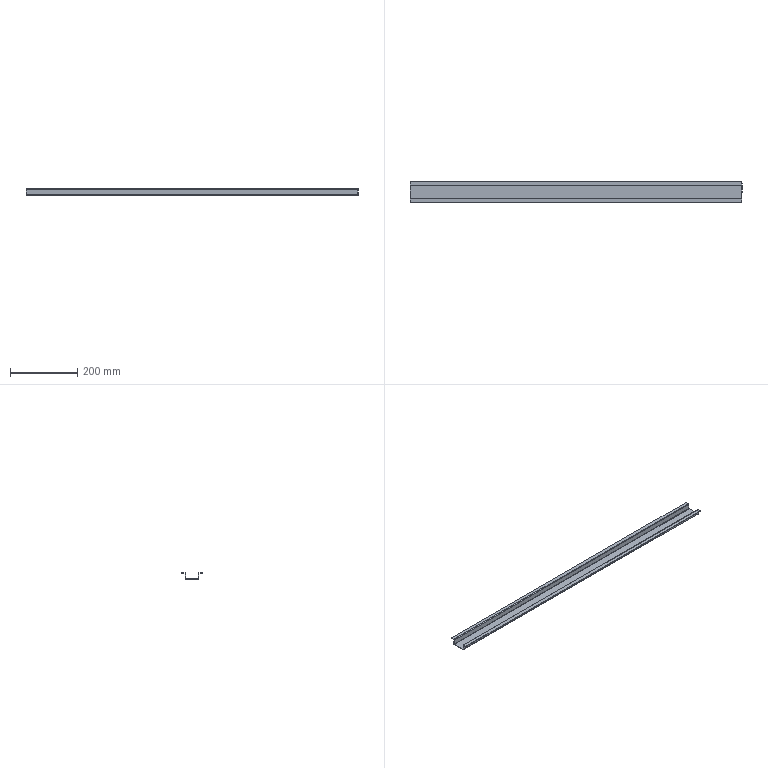Component | SolidWorks | AirFurnaceElectricalCabinet-DoorPanelAssembly-1_DoorPanelReinforcementPlate-L790-1 | 1 solid | 38 faces | box 990 x 61.6 x 18 mm | volume 110344 mm3 | plane 30 | cylinder 8 | commonest cylinder face diameters 3.9 x4 1.5 x4
STEP:
#1=CARTESIAN_POINT('',(-19.488,27.38,9.272));
#2=VERTEX_POINT('',#1);
#3=CARTESIAN_POINT('',(-19.488,28.801,9.272));
#4=VERTEX_POINT('',#3);
#5=CARTESIAN_POINT('',(-19.488,27.303,9.272));
#6=DIRECTION('',(0.,1.,0.));
#7=VECTOR('',#6,39.37);
#8=LINE('',#5,#7);
#9=EDGE_CURVE('',#2,#4,#8,.T.);
#10=ORIENTED_EDGE('',*,*,#9,.F.);
#11=CARTESIAN_POINT('',(-19.488,27.38,9.319));
#12=VERTEX_POINT('',#11);
#13=CARTESIAN_POINT('',(-19.488,27.38,9.272));
#14=DIRECTION('',(0.,-0.,1.));
#15=VECTOR('',#14,39.37);
#16=LINE('',#13,#15);
#17=EDGE_CURVE('',#2,#12,#16,.T.);
#18=ORIENTED_EDGE('',*,*,#17,.T.);
#19=CARTESIAN_POINT('',(-19.488,28.801,9.319));
#20=VERTEX_POINT('',#19);
#21=CARTESIAN_POINT('',(-19.488,27.303,9.319));
#22=DIRECTION('',(0.,1.,0.));
#23=VECTOR('',#22,39.37);
#24=LINE('',#21,#23);
#25=EDGE_CURVE('',#12,#20,#24,.T.);
#26=ORIENTED_EDGE('',*,*,#25,.T.);
#27=CARTESIAN_POINT('',(-19.488,28.801,9.319));
#28=DIRECTION('',(0.,0.,-1.));
#29=VECTOR('',#28,39.37);
#30=LINE('',#27,#29);
#31=EDGE_CURVE('',#20,#4,#30,.T.);
#32=ORIENTED_EDGE('',*,*,#31,.T.);
#33=EDGE_LOOP('',(#10,#18,#26,#32));
#34=FACE_OUTER_BOUND('',#33,.T.);
#35=CARTESIAN_POINT('',(-19.488,27.35,9.348));
#36=DIRECTION('',(-1.,0.,0.));
#37=DIRECTION('',(0.,1.,0.));
#38=AXIS2_PLACEMENT_3D('',#35,#36,#37);
#39=PLANE('',#38);
#40=ADVANCED_FACE('',(#34),#39,.T.);
#41=CARTESIAN_POINT('',(19.488,27.38,9.272));
#42=VERTEX_POINT('',#41);
#43=CARTESIAN_POINT('',(19.488,28.801,9.272));
#44=VERTEX_POINT('',#43);
#45=CARTESIAN_POINT('',(19.488,27.303,9.272));
#46=DIRECTION('',(0.,1.,0.));
#47=VECTOR('',#46,39.37);
#48=LINE('',#45,#47);
#49=EDGE_CURVE('',#42,#44,#48,.T.);
#50=ORIENTED_EDGE('',*,*,#49,.T.);
#51=CARTESIAN_POINT('',(19.488,28.801,9.319));
#52=VERTEX_POINT('',#51);
#53=CARTESIAN_POINT('',(19.488,28.801,9.272));
#54=DIRECTION('',(0.,-0.,1.));
#55=VECTOR('',#54,39.37);
#56=LINE('',#53,#55);
#57=EDGE_CURVE('',#44,#52,#56,.T.);
#58=ORIENTED_EDGE('',*,*,#57,.T.);
#59=CARTESIAN_POINT('',(19.488,27.38,9.319));
#60=VERTEX_POINT('',#59);
#61=CARTESIAN_POINT('',(19.488,27.303,9.319));
#62=DIRECTION('',(0.,1.,0.));
#63=VECTOR('',#62,39.37);
#64=LINE('',#61,#63);
#65=EDGE_CURVE('',#60,#52,#64,.T.);
#66=ORIENTED_EDGE('',*,*,#65,.F.);
#67=CARTESIAN_POINT('',(19.488,27.38,9.319));
#68=DIRECTION('',(0.,0.,-1.));
#69=VECTOR('',#68,39.37);
#70=LINE('',#67,#69);
#71=EDGE_CURVE('',#60,#42,#70,.T.);
#72=ORIENTED_EDGE('',*,*,#71,.T.);
#73=EDGE_LOOP('',(#50,#58,#66,#72));
#74=FACE_OUTER_BOUND('',#73,.T.);
#75=CARTESIAN_POINT('',(19.488,28.831,9.348));
#76=DIRECTION('',(1.,-0.,0.));
#77=DIRECTION('',(-0.,-1.,-0.));
#78=AXIS2_PLACEMENT_3D('',#75,#76,#77);
#79=PLANE('',#78);
#80=ADVANCED_FACE('',(#74),#79,.T.);
#81=ORIENTED_EDGE('',*,*,#49,.F.);
#82=CARTESIAN_POINT('',(-19.488,27.38,9.272));
#83=DIRECTION('',(1.,-0.,0.));
#84=VECTOR('',#83,39.37);
#85=LINE('',#82,#84);
#86=EDGE_CURVE('',#2,#42,#85,.T.);
#87=ORIENTED_EDGE('',*,*,#86,.F.);
#88=ORIENTED_EDGE('',*,*,#9,.T.);
#89=CARTESIAN_POINT('',(-19.488,28.801,9.272));
#90=DIRECTION('',(1.,-0.,0.));
#91=VECTOR('',#90,39.37);
#92=LINE('',#89,#91);
#93=EDGE_CURVE('',#4,#44,#92,.T.);
#94=ORIENTED_EDGE('',*,*,#93,.T.);
#95=EDGE_LOOP('',(#81,#87,#88,#94));
#96=FACE_OUTER_BOUND('',#95,.T.);
#97=CARTESIAN_POINT('',(-19.488,27.303,9.272));
#98=DIRECTION('',(0.,0.,-1.));
#99=DIRECTION('',(-0.,-1.,-0.));
#100=AXIS2_PLACEMENT_3D('',#97,#98,#99);
#101=PLANE('',#100);
#102=ADVANCED_FACE('',(#96),#101,.T.);
#103=ORIENTED_EDGE('',*,*,#65,.T.);
#104=CARTESIAN_POINT('',(-19.488,28.801,9.319));
#105=DIRECTION('',(1.,-0.,0.));
#106=VECTOR('',#105,39.37);
#107=LINE('',#104,#106);
#108=EDGE_CURVE('',#20,#52,#107,.T.);
#109=ORIENTED_EDGE('',*,*,#108,.F.);
#110=ORIENTED_EDGE('',*,*,#25,.F.);
#111=CARTESIAN_POINT('',(-19.488,27.38,9.319));
#112=DIRECTION('',(1.,-0.,0.));
#113=VECTOR('',#112,39.37);
#114=LINE('',#111,#113);
#115=EDGE_CURVE('',#12,#60,#114,.T.);
#116=ORIENTED_EDGE('',*,*,#115,.T.);
#117=EDGE_LOOP('',(#103,#109,#110,#116));
#118=FACE_OUTER_BOUND('',#117,.T.);
#119=CARTESIAN_POINT('',(-19.488,27.303,9.319));
#120=DIRECTION('',(0.,0.,-1.));
#121=DIRECTION('',(-0.,-1.,-0.));
#122=AXIS2_PLACEMENT_3D('',#119,#120,#121);
#123=PLANE('',#122);
#124=ADVANCED_FACE('',(#118),#123,.F.);
#125=ORIENTED_EDGE('',*,*,#31,.F.);
#126=CARTESIAN_POINT('',(-19.488,28.831,9.348));
#127=VERTEX_POINT('',#126);
#128=CARTESIAN_POINT('',(-19.488,28.801,9.348));
#129=DIRECTION('',(1.,-0.,0.));
#130=DIRECTION('',(0.,-1.,0.));
#131=AXIS2_PLACEMENT_3D('',#128,#129,#130);
#132=CIRCLE('',#131,0.02953);
#133=EDGE_CURVE('',#20,#127,#132,.T.);
#134=ORIENTED_EDGE('',*,*,#133,.T.);
#135=CARTESIAN_POINT('',(-19.488,28.878,9.348));
#136=VERTEX_POINT('',#135);
#137=CARTESIAN_POINT('',(-19.488,28.878,9.348));
#138=DIRECTION('',(-0.,-1.,-0.));
#139=VECTOR('',#138,39.37);
#140=LINE('',#137,#139);
#141=EDGE_CURVE('',#136,#127,#140,.T.);
#142=ORIENTED_EDGE('',*,*,#141,.F.);
#143=CARTESIAN_POINT('',(-19.488,28.801,9.348));
#144=DIRECTION('',(1.,-0.,0.));
#145=DIRECTION('',(0.,-1.,0.));
#146=AXIS2_PLACEMENT_3D('',#143,#144,#145);
#147=CIRCLE('',#146,0.07677);
#148=EDGE_CURVE('',#4,#136,#147,.T.);
#149=ORIENTED_EDGE('',*,*,#148,.F.);
#150=EDGE_LOOP('',(#125,#134,#142,#149));
#151=FACE_OUTER_BOUND('',#150,.T.);
#152=CARTESIAN_POINT('',(-19.488,28.801,9.348));
#153=DIRECTION('',(-1.,0.,0.));
#154=DIRECTION('',(0.,1.,0.));
#155=AXIS2_PLACEMENT_3D('',#152,#153,#154);
#156=PLANE('',#155);
#157=ADVANCED_FACE('',(#151),#156,.T.);
#158=CARTESIAN_POINT('',(19.488,28.831,9.348));
#159=VERTEX_POINT('',#158);
#160=CARTESIAN_POINT('',(19.488,28.878,9.348));
#161=VERTEX_POINT('',#160);
#162=CARTESIAN_POINT('',(19.488,28.831,9.348));
#163=DIRECTION('',(0.,1.,0.));
#164=VECTOR('',#163,39.37);
#165=LINE('',#162,#164);
#166=EDGE_CURVE('',#159,#161,#165,.T.);
#167=ORIENTED_EDGE('',*,*,#166,.F.);
#168=CARTESIAN_POINT('',(19.488,28.801,9.348));
#169=DIRECTION('',(-1.,0.,0.));
#170=DIRECTION('',(0.,-1.,0.));
#171=AXIS2_PLACEMENT_3D('',#168,#169,#170);
#172=CIRCLE('',#171,0.02953);
#173=EDGE_CURVE('',#159,#52,#172,.T.);
#174=ORIENTED_EDGE('',*,*,#173,.T.);
#175=ORIENTED_EDGE('',*,*,#57,.F.);
#176=CARTESIAN_POINT('',(19.488,28.801,9.348));
#177=DIRECTION('',(-1.,0.,0.));
#178=DIRECTION('',(0.,1.,0.));
#179=AXIS2_PLACEMENT_3D('',#176,#177,#178);
#180=CIRCLE('',#179,0.07677);
#181=EDGE_CURVE('',#161,#44,#180,.T.);
#182=ORIENTED_EDGE('',*,*,#181,.F.);
#183=EDGE_LOOP('',(#167,#174,#175,#182));
#184=FACE_OUTER_BOUND('',#183,.T.);
#185=CARTESIAN_POINT('',(19.488,28.801,9.348));
#186=DIRECTION('',(1.,-0.,0.));
#187=DIRECTION('',(-0.,-1.,-0.));
#188=AXIS2_PLACEMENT_3D('',#185,#186,#187);
#189=PLANE('',#188);
#190=ADVANCED_FACE('',(#184),#189,.T.);
#191=ORIENTED_EDGE('',*,*,#181,.T.);
#192=ORIENTED_EDGE('',*,*,#93,.F.);
#193=ORIENTED_EDGE('',*,*,#148,.T.);
#194=CARTESIAN_POINT('',(-19.488,28.878,9.348));
#195=DIRECTION('',(1.,-0.,0.));
#196=VECTOR('',#195,39.37);
#197=LINE('',#194,#196);
#198=EDGE_CURVE('',#136,#161,#197,.T.);
#199=ORIENTED_EDGE('',*,*,#198,.T.);
#200=EDGE_LOOP('',(#191,#192,#193,#199));
#201=FACE_OUTER_BOUND('',#200,.T.);
#202=CARTESIAN_POINT('',(-38.976,28.801,9.348));
#203=DIRECTION('',(1.,-0.,0.));
#204=DIRECTION('',(0.,-1.,0.));
#205=AXIS2_PLACEMENT_3D('',#202,#203,#204);
#206=CYLINDRICAL_SURFACE('',#205,0.07677);
#207=ADVANCED_FACE('',(#201),#206,.T.);
#208=ORIENTED_EDGE('',*,*,#173,.F.);
#209=CARTESIAN_POINT('',(-19.488,28.831,9.348));
#210=DIRECTION('',(1.,-0.,0.));
#211=VECTOR('',#210,39.37);
#212=LINE('',#209,#211);
#213=EDGE_CURVE('',#127,#159,#212,.T.);
#214=ORIENTED_EDGE('',*,*,#213,.F.);
#215=ORIENTED_EDGE('',*,*,#133,.F.);
#216=ORIENTED_EDGE('',*,*,#108,.T.);
#217=EDGE_LOOP('',(#208,#214,#215,#216));
#218=FACE_OUTER_BOUND('',#217,.T.);
#219=CARTESIAN_POINT('',(-38.976,28.801,9.348));
#220=DIRECTION('',(1.,-0.,0.));
#221=DIRECTION('',(0.,-1.,0.));
#222=AXIS2_PLACEMENT_3D('',#219,#220,#221);
#223=CYLINDRICAL_SURFACE('',#222,0.02953);
#224=ADVANCED_FACE('',(#218),#223,.F.);
#225=CARTESIAN_POINT('',(19.488,29.303,9.933));
#226=VERTEX_POINT('',#225);
#227=CARTESIAN_POINT('',(19.488,29.303,9.98));
#228=VERTEX_POINT('',#227);
#229=CARTESIAN_POINT('',(19.488,29.303,9.933));
#230=DIRECTION('',(0.,-0.,1.));
#231=VECTOR('',#230,39.37);
#232=LINE('',#229,#231);
#233=EDGE_CURVE('',#226,#228,#232,.T.);
#234=ORIENTED_EDGE('',*,*,#233,.F.);
#235=CARTESIAN_POINT('',(-19.488,29.303,9.933));
#236=VERTEX_POINT('',#235);
#237=CARTESIAN_POINT('',(-19.488,29.303,9.933));
#238=DIRECTION('',(1.,-0.,0.));
#239=VECTOR('',#238,39.37);
#240=LINE('',#237,#239);
#241=EDGE_CURVE('',#236,#226,#240,.T.);
#242=ORIENTED_EDGE('',*,*,#241,.F.);
#243=CARTESIAN_POINT('',(-19.488,29.303,9.98));
#244=VERTEX_POINT('',#243);
#245=CARTESIAN_POINT('',(-19.488,29.303,9.933));
#246=DIRECTION('',(0.,-0.,1.));
#247=VECTOR('',#246,39.37);
#248=LINE('',#245,#247);
#249=EDGE_CURVE('',#236,#244,#248,.T.);
#250=ORIENTED_EDGE('',*,*,#249,.T.);
#251=CARTESIAN_POINT('',(-19.488,29.303,9.98));
#252=DIRECTION('',(1.,-0.,0.));
#253=VECTOR('',#252,39.37);
#254=LINE('',#251,#253);
#255=EDGE_CURVE('',#244,#228,#254,.T.);
#256=ORIENTED_EDGE('',*,*,#255,.T.);
#257=EDGE_LOOP('',(#234,#242,#250,#256));
#258=FACE_OUTER_BOUND('',#257,.T.);
#259=CARTESIAN_POINT('',(-19.488,29.303,9.933));
#260=DIRECTION('',(0.,1.,0.));
#261=DIRECTION('',(1.,-0.,0.));
#262=AXIS2_PLACEMENT_3D('',#259,#260,#261);
#263=PLANE('',#262);
#264=ADVANCED_FACE('',(#258),#263,.T.);
#265=CARTESIAN_POINT('',(19.488,28.907,9.98));
#266=VERTEX_POINT('',#265);
#267=CARTESIAN_POINT('',(19.488,28.878,9.98));
#268=DIRECTION('',(0.,1.,0.));
#269=VECTOR('',#268,39.37);
#270=LINE('',#267,#269);
#271=EDGE_CURVE('',#266,#228,#270,.T.);
#272=ORIENTED_EDGE('',*,*,#271,.F.);
#273=CARTESIAN_POINT('',(19.488,28.907,9.933));
#274=VERTEX_POINT('',#273);
#275=CARTESIAN_POINT('',(19.488,28.907,9.98));
#276=DIRECTION('',(0.,0.,-1.));
#277=VECTOR('',#276,39.37);
#278=LINE('',#275,#277);
#279=EDGE_CURVE('',#266,#274,#278,.T.);
#280=ORIENTED_EDGE('',*,*,#279,.T.);
#281=CARTESIAN_POINT('',(19.488,28.878,9.933));
#282=DIRECTION('',(0.,1.,0.));
#283=VECTOR('',#282,39.37);
#284=LINE('',#281,#283);
#285=EDGE_CURVE('',#274,#226,#284,.T.);
#286=ORIENTED_EDGE('',*,*,#285,.T.);
#287=ORIENTED_EDGE('',*,*,#233,.T.);
#288=EDGE_LOOP('',(#272,#280,#286,#287));
#289=FACE_OUTER_BOUND('',#288,.T.);
#290=CARTESIAN_POINT('',(19.488,28.907,9.904));
#291=DIRECTION('',(1.,-0.,0.));
#292=DIRECTION('',(-0.,-1.,-0.));
#293=AXIS2_PLACEMENT_3D('',#290,#291,#292);
#294=PLANE('',#293);
#295=ADVANCED_FACE('',(#289),#294,.T.);
#296=ORIENTED_EDGE('',*,*,#271,.T.);
#297=ORIENTED_EDGE('',*,*,#255,.F.);
#298=CARTESIAN_POINT('',(-19.488,28.907,9.98));
#299=VERTEX_POINT('',#298);
#300=CARTESIAN_POINT('',(-19.488,28.878,9.98));
#301=DIRECTION('',(0.,1.,0.));
#302=VECTOR('',#301,39.37);
#303=LINE('',#300,#302);
#304=EDGE_CURVE('',#299,#244,#303,.T.);
#305=ORIENTED_EDGE('',*,*,#304,.F.);
#306=CARTESIAN_POINT('',(-19.488,28.907,9.98));
#307=DIRECTION('',(1.,-0.,0.));
#308=VECTOR('',#307,39.37);
#309=LINE('',#306,#308);
#310=EDGE_CURVE('',#299,#266,#309,.T.);
#311=ORIENTED_EDGE('',*,*,#310,.T.);
#312=EDGE_LOOP('',(#296,#297,#305,#311));
#313=FACE_OUTER_BOUND('',#312,.T.);
#314=CARTESIAN_POINT('',(-19.488,28.878,9.98));
#315=DIRECTION('',(0.,0.,-1.));
#316=DIRECTION('',(-0.,-1.,-0.));
#317=AXIS2_PLACEMENT_3D('',#314,#315,#316);
#318=PLANE('',#317);
#319=ADVANCED_FACE('',(#313),#318,.F.);
#320=CARTESIAN_POINT('',(-19.488,28.907,9.933));
#321=VERTEX_POINT('',#320);
#322=CARTESIAN_POINT('',(-19.488,28.878,9.933));
#323=DIRECTION('',(0.,1.,0.));
#324=VECTOR('',#323,39.37);
#325=LINE('',#322,#324);
#326=EDGE_CURVE('',#321,#236,#325,.T.);
#327=ORIENTED_EDGE('',*,*,#326,.F.);
#328=CARTESIAN_POINT('',(-19.488,28.907,9.933));
#329=DIRECTION('',(0.,-0.,1.));
#330=VECTOR('',#329,39.37);
#331=LINE('',#328,#330);
#332=EDGE_CURVE('',#321,#299,#331,.T.);
#333=ORIENTED_EDGE('',*,*,#332,.T.);
#334=ORIENTED_EDGE('',*,*,#304,.T.);
#335=ORIENTED_EDGE('',*,*,#249,.F.);
#336=EDGE_LOOP('',(#327,#333,#334,#335));
#337=FACE_OUTER_BOUND('',#336,.T.);
#338=CARTESIAN_POINT('',(-19.488,28.831,9.904));
#339=DIRECTION('',(-1.,0.,0.));
#340=DIRECTION('',(0.,1.,0.));
#341=AXIS2_PLACEMENT_3D('',#338,#339,#340);
#342=PLANE('',#341);
#343=ADVANCED_FACE('',(#337),#342,.T.);
#344=ORIENTED_EDGE('',*,*,#285,.F.);
#345=CARTESIAN_POINT('',(-19.488,28.907,9.933));
#346=DIRECTION('',(1.,-0.,0.));
#347=VECTOR('',#346,39.37);
#348=LINE('',#345,#347);
#349=EDGE_CURVE('',#321,#274,#348,.T.);
#350=ORIENTED_EDGE('',*,*,#349,.F.);
#351=ORIENTED_EDGE('',*,*,#326,.T.);
#352=ORIENTED_EDGE('',*,*,#241,.T.);
#353=EDGE_LOOP('',(#344,#350,#351,#352));
#354=FACE_OUTER_BOUND('',#353,.T.);
#355=CARTESIAN_POINT('',(-19.488,28.878,9.933));
#356=DIRECTION('',(0.,0.,-1.));
#357=DIRECTION('',(-0.,-1.,-0.));
#358=AXIS2_PLACEMENT_3D('',#355,#356,#357);
#359=PLANE('',#358);
#360=ADVANCED_FACE('',(#354),#359,.T.);
#361=ORIENTED_EDGE('',*,*,#279,.F.);
#362=CARTESIAN_POINT('',(19.488,28.831,9.904));
#363=VERTEX_POINT('',#362);
#364=CARTESIAN_POINT('',(19.488,28.907,9.904));
#365=DIRECTION('',(1.,-0.,0.));
#366=DIRECTION('',(0.,0.,-1.));
#367=AXIS2_PLACEMENT_3D('',#364,#365,#366);
#368=CIRCLE('',#367,0.07677);
#369=EDGE_CURVE('',#266,#363,#368,.T.);
#370=ORIENTED_EDGE('',*,*,#369,.T.);
#371=CARTESIAN_POINT('',(19.488,28.878,9.904));
#372=VERTEX_POINT('',#371);
#373=CARTESIAN_POINT('',(19.488,28.878,9.904));
#374=DIRECTION('',(-0.,-1.,-0.));
#375=VECTOR('',#374,39.37);
#376=LINE('',#373,#375);
#377=EDGE_CURVE('',#372,#363,#376,.T.);
#378=ORIENTED_EDGE('',*,*,#377,.F.);
#379=CARTESIAN_POINT('',(19.488,28.907,9.904));
#380=DIRECTION('',(1.,-0.,0.));
#381=DIRECTION('',(0.,0.,-1.));
#382=AXIS2_PLACEMENT_3D('',#379,#380,#381);
#383=CIRCLE('',#382,0.02953);
#384=EDGE_CURVE('',#274,#372,#383,.T.);
#385=ORIENTED_EDGE('',*,*,#384,.F.);
#386=EDGE_LOOP('',(#361,#370,#378,#385));
#387=FACE_OUTER_BOUND('',#386,.T.);
#388=CARTESIAN_POINT('',(19.488,28.907,9.904));
#389=DIRECTION('',(-1.,0.,0.));
#390=DIRECTION('',(0.,0.,1.));
#391=AXIS2_PLACEMENT_3D('',#388,#389,#390);
#392=PLANE('',#391);
#393=ADVANCED_FACE('',(#387),#392,.F.);
#394=ORIENTED_EDGE('',*,*,#369,.F.);
#395=ORIENTED_EDGE('',*,*,#310,.F.);
#396=CARTESIAN_POINT('',(-19.488,28.831,9.904));
#397=VERTEX_POINT('',#396);
#398=CARTESIAN_POINT('',(-19.488,28.907,9.904));
#399=DIRECTION('',(-1.,0.,0.));
#400=DIRECTION('',(0.,0.,-1.));
#401=AXIS2_PLACEMENT_3D('',#398,#399,#400);
#402=CIRCLE('',#401,0.07677);
#403=EDGE_CURVE('',#397,#299,#402,.T.);
#404=ORIENTED_EDGE('',*,*,#403,.F.);
#405=CARTESIAN_POINT('',(-19.488,28.831,9.904));
#406=DIRECTION('',(1.,-0.,0.));
#407=VECTOR('',#406,39.37);
#408=LINE('',#405,#407);
#409=EDGE_CURVE('',#397,#363,#408,.T.);
#410=ORIENTED_EDGE('',*,*,#409,.T.);
#411=EDGE_LOOP('',(#394,#395,#404,#410));
#412=FACE_OUTER_BOUND('',#411,.T.);
#413=CARTESIAN_POINT('',(-38.976,28.907,9.904));
#414=DIRECTION('',(1.,-0.,0.));
#415=DIRECTION('',(0.,0.,-1.));
#416=AXIS2_PLACEMENT_3D('',#413,#414,#415);
#417=CYLINDRICAL_SURFACE('',#416,0.07677);
#418=ADVANCED_FACE('',(#412),#417,.T.);
#419=CARTESIAN_POINT('',(-19.488,28.878,9.904));
#420=VERTEX_POINT('',#419);
#421=CARTESIAN_POINT('',(-19.488,28.831,9.904));
#422=DIRECTION('',(0.,1.,0.));
#423=VECTOR('',#422,39.37);
#424=LINE('',#421,#423);
#425=EDGE_CURVE('',#397,#420,#424,.T.);
#426=ORIENTED_EDGE('',*,*,#425,.F.);
#427=ORIENTED_EDGE('',*,*,#403,.T.);
#428=ORIENTED_EDGE('',*,*,#332,.F.);
#429=CARTESIAN_POINT('',(-19.488,28.907,9.904));
#430=DIRECTION('',(-1.,0.,0.));
#431=DIRECTION('',(0.,0.,1.));
#432=AXIS2_PLACEMENT_3D('',#429,#430,#431);
#433=CIRCLE('',#432,0.02953);
#434=EDGE_CURVE('',#420,#321,#433,.T.);
#435=ORIENTED_EDGE('',*,*,#434,.F.);
#436=EDGE_LOOP('',(#426,#427,#428,#435));
#437=FACE_OUTER_BOUND('',#436,.T.);
#438=CARTESIAN_POINT('',(-19.488,28.907,9.904));
#439=DIRECTION('',(1.,-0.,-0.));
#440=DIRECTION('',(-0.,-0.,-1.));
#441=AXIS2_PLACEMENT_3D('',#438,#439,#440);
#442=PLANE('',#441);
#443=ADVANCED_FACE('',(#437),#442,.F.);
#444=ORIENTED_EDGE('',*,*,#384,.T.);
#445=CARTESIAN_POINT('',(-19.488,28.878,9.904));
#446=DIRECTION('',(1.,-0.,0.));
#447=VECTOR('',#446,39.37);
#448=LINE('',#445,#447);
#449=EDGE_CURVE('',#420,#372,#448,.T.);
#450=ORIENTED_EDGE('',*,*,#449,.F.);
#451=ORIENTED_EDGE('',*,*,#434,.T.);
#452=ORIENTED_EDGE('',*,*,#349,.T.);
#453=EDGE_LOOP('',(#444,#450,#451,#452));
#454=FACE_OUTER_BOUND('',#453,.T.);
#455=CARTESIAN_POINT('',(-38.976,28.907,9.904));
#456=DIRECTION('',(1.,-0.,0.));
#457=DIRECTION('',(0.,0.,-1.));
#458=AXIS2_PLACEMENT_3D('',#455,#456,#457);
#459=CYLINDRICAL_SURFACE('',#458,0.02953);
#460=ADVANCED_FACE('',(#454),#459,.F.);
#461=CARTESIAN_POINT('',(19.488,28.878,9.272));
#462=DIRECTION('',(0.,-0.,1.));
#463=VECTOR('',#462,39.37);
#464=LINE('',#461,#463);
#465=EDGE_CURVE('',#161,#372,#464,.T.);
#466=ORIENTED_EDGE('',*,*,#465,.F.);
#467=ORIENTED_EDGE('',*,*,#198,.F.);
#468=CARTESIAN_POINT('',(-19.488,28.878,9.272));
#469=DIRECTION('',(0.,-0.,1.));
#470=VECTOR('',#469,39.37);
#471=LINE('',#468,#470);
#472=EDGE_CURVE('',#136,#420,#471,.T.);
#473=ORIENTED_EDGE('',*,*,#472,.T.);
#474=ORIENTED_EDGE('',*,*,#449,.T.);
#475=EDGE_LOOP('',(#466,#467,#473,#474));
#476=FACE_OUTER_BOUND('',#475,.T.);
#477=CARTESIAN_POINT('',(-19.488,28.878,9.272));
#478=DIRECTION('',(0.,1.,0.));
#479=DIRECTION('',(1.,-0.,0.));
#480=AXIS2_PLACEMENT_3D('',#477,#478,#479);
#481=PLANE('',#480);
#482=ADVANCED_FACE('',(#476),#481,.T.);
#483=ORIENTED_EDGE('',*,*,#472,.F.);
#484=ORIENTED_EDGE('',*,*,#141,.T.);
#485=CARTESIAN_POINT('',(-19.488,28.831,9.272));
#486=DIRECTION('',(0.,-0.,1.));
#487=VECTOR('',#486,39.37);
#488=LINE('',#485,#487);
#489=EDGE_CURVE('',#127,#397,#488,.T.);
#490=ORIENTED_EDGE('',*,*,#489,.T.);
#491=ORIENTED_EDGE('',*,*,#425,.T.);
#492=EDGE_LOOP('',(#483,#484,#490,#491));
#493=FACE_OUTER_BOUND('',#492,.T.);
#494=CARTESIAN_POINT('',(-19.488,28.801,9.319));
#495=DIRECTION('',(-1.,0.,0.));
#496=DIRECTION('',(0.,1.,0.));
#497=AXIS2_PLACEMENT_3D('',#494,#495,#496);
#498=PLANE('',#497);
#499=ADVANCED_FACE('',(#493),#498,.T.);
#500=CARTESIAN_POINT('',(19.488,28.831,9.272));
#501=DIRECTION('',(0.,-0.,1.));
#502=VECTOR('',#501,39.37);
#503=LINE('',#500,#502);
#504=EDGE_CURVE('',#159,#363,#503,.T.);
#505=ORIENTED_EDGE('',*,*,#504,.T.);
#506=ORIENTED_EDGE('',*,*,#409,.F.);
#507=ORIENTED_EDGE('',*,*,#489,.F.);
#508=ORIENTED_EDGE('',*,*,#213,.T.);
#509=EDGE_LOOP('',(#505,#506,#507,#508));
#510=FACE_OUTER_BOUND('',#509,.T.);
#511=CARTESIAN_POINT('',(-19.488,28.831,9.272));
#512=DIRECTION('',(0.,1.,0.));
#513=DIRECTION('',(1.,-0.,0.));
#514=AXIS2_PLACEMENT_3D('',#511,#512,#513);
#515=PLANE('',#514);
#516=ADVANCED_FACE('',(#510),#515,.F.);
#517=ORIENTED_EDGE('',*,*,#465,.T.);
#518=ORIENTED_EDGE('',*,*,#377,.T.);
#519=ORIENTED_EDGE('',*,*,#504,.F.);
#520=ORIENTED_EDGE('',*,*,#166,.T.);
#521=EDGE_LOOP('',(#517,#518,#519,#520));
#522=FACE_OUTER_BOUND('',#521,.T.);
#523=CARTESIAN_POINT('',(19.488,28.907,9.98));
#524=DIRECTION('',(1.,-0.,0.));
#525=DIRECTION('',(-0.,-1.,-0.));
#526=AXIS2_PLACEMENT_3D('',#523,#524,#525);
#527=PLANE('',#526);
#528=ADVANCED_FACE('',(#522),#527,.T.);
#529=CARTESIAN_POINT('',(-19.488,27.35,9.348));
#530=VERTEX_POINT('',#529);
#531=CARTESIAN_POINT('',(-19.488,27.303,9.348));
#532=VERTEX_POINT('',#531);
#533=CARTESIAN_POINT('',(-19.488,27.35,9.348));
#534=DIRECTION('',(-0.,-1.,-0.));
#535=VECTOR('',#534,39.37);
#536=LINE('',#533,#535);
#537=EDGE_CURVE('',#530,#532,#536,.T.);
#538=ORIENTED_EDGE('',*,*,#537,.F.);
#539=CARTESIAN_POINT('',(-19.488,27.38,9.348));
#540=DIRECTION('',(1.,-0.,0.));
#541=DIRECTION('',(0.,1.,0.));
#542=AXIS2_PLACEMENT_3D('',#539,#540,#541);
#543=CIRCLE('',#542,0.02953);
#544=EDGE_CURVE('',#530,#12,#543,.T.);
#545=ORIENTED_EDGE('',*,*,#544,.T.);
#546=ORIENTED_EDGE('',*,*,#17,.F.);
#547=CARTESIAN_POINT('',(-19.488,27.38,9.348));
#548=DIRECTION('',(1.,-0.,0.));
#549=DIRECTION('',(0.,-1.,0.));
#550=AXIS2_PLACEMENT_3D('',#547,#548,#549);
#551=CIRCLE('',#550,0.07677);
#552=EDGE_CURVE('',#532,#2,#551,.T.);
#553=ORIENTED_EDGE('',*,*,#552,.F.);
#554=EDGE_LOOP('',(#538,#545,#546,#553));
#555=FACE_OUTER_BOUND('',#554,.T.);
#556=CARTESIAN_POINT('',(-19.488,27.38,9.348));
#557=DIRECTION('',(-1.,0.,0.));
#558=DIRECTION('',(0.,1.,0.));
#559=AXIS2_PLACEMENT_3D('',#556,#557,#558);
#560=PLANE('',#559);
#561=ADVANCED_FACE('',(#555),#560,.T.);
#562=ORIENTED_EDGE('',*,*,#71,.F.);
#563=CARTESIAN_POINT('',(19.488,27.35,9.348));
#564=VERTEX_POINT('',#563);
#565=CARTESIAN_POINT('',(19.488,27.38,9.348));
#566=DIRECTION('',(-1.,0.,0.));
#567=DIRECTION('',(0.,1.,0.));
#568=AXIS2_PLACEMENT_3D('',#565,#566,#567);
#569=CIRCLE('',#568,0.02953);
#570=EDGE_CURVE('',#60,#564,#569,.T.);
#571=ORIENTED_EDGE('',*,*,#570,.T.);
#572=CARTESIAN_POINT('',(19.488,27.303,9.348));
#573=VERTEX_POINT('',#572);
#574=CARTESIAN_POINT('',(19.488,27.303,9.348));
#575=DIRECTION('',(0.,1.,0.));
#576=VECTOR('',#575,39.37);
#577=LINE('',#574,#576);
#578=EDGE_CURVE('',#573,#564,#577,.T.);
#579=ORIENTED_EDGE('',*,*,#578,.F.);
#580=CARTESIAN_POINT('',(19.488,27.38,9.348));
#581=DIRECTION('',(-1.,0.,0.));
#582=DIRECTION('',(0.,1.,0.));
#583=AXIS2_PLACEMENT_3D('',#580,#581,#582);
#584=CIRCLE('',#583,0.07677);
#585=EDGE_CURVE('',#42,#573,#584,.T.);
#586=ORIENTED_EDGE('',*,*,#585,.F.);
#587=EDGE_LOOP('',(#562,#571,#579,#586));
#588=FACE_OUTER_BOUND('',#587,.T.);
#589=CARTESIAN_POINT('',(19.488,27.38,9.348));
#590=DIRECTION('',(1.,-0.,0.));
#591=DIRECTION('',(-0.,-1.,-0.));
#592=AXIS2_PLACEMENT_3D('',#589,#590,#591);
#593=PLANE('',#592);
#594=ADVANCED_FACE('',(#588),#593,.T.);
#595=ORIENTED_EDGE('',*,*,#585,.T.);
#596=CARTESIAN_POINT('',(-19.488,27.303,9.348));
#597=DIRECTION('',(1.,-0.,0.));
#598=VECTOR('',#597,39.37);
#599=LINE('',#596,#598);
#600=EDGE_CURVE('',#532,#573,#599,.T.);
#601=ORIENTED_EDGE('',*,*,#600,.F.);
#602=ORIENTED_EDGE('',*,*,#552,.T.);
#603=ORIENTED_EDGE('',*,*,#86,.T.);
#604=EDGE_LOOP('',(#595,#601,#602,#603));
#605=FACE_OUTER_BOUND('',#604,.T.);
#606=CARTESIAN_POINT('',(38.976,27.38,9.348));
#607=DIRECTION('',(-1.,0.,0.));
#608=DIRECTION('',(0.,1.,0.));
#609=AXIS2_PLACEMENT_3D('',#606,#607,#608);
#610=CYLINDRICAL_SURFACE('',#609,0.07677);
#611=ADVANCED_FACE('',(#605),#610,.T.);
#612=ORIENTED_EDGE('',*,*,#570,.F.);
#613=ORIENTED_EDGE('',*,*,#115,.F.);
#614=ORIENTED_EDGE('',*,*,#544,.F.);
#615=CARTESIAN_POINT('',(-19.488,27.35,9.348));
#616=DIRECTION('',(1.,-0.,0.));
#617=VECTOR('',#616,39.37);
#618=LINE('',#615,#617);
#619=EDGE_CURVE('',#530,#564,#618,.T.);
#620=ORIENTED_EDGE('',*,*,#619,.T.);
#621=EDGE_LOOP('',(#612,#613,#614,#620));
#622=FACE_OUTER_BOUND('',#621,.T.);
#623=CARTESIAN_POINT('',(38.976,27.38,9.348));
#624=DIRECTION('',(-1.,0.,0.));
#625=DIRECTION('',(0.,1.,0.));
#626=AXIS2_PLACEMENT_3D('',#623,#624,#625);
#627=CYLINDRICAL_SURFACE('',#626,0.02953);
#628=ADVANCED_FACE('',(#622),#627,.F.);
#629=CARTESIAN_POINT('',(19.488,27.303,9.904));
#630=VERTEX_POINT('',#629);
#631=CARTESIAN_POINT('',(19.488,27.303,9.933));
#632=DIRECTION('',(0.,0.,-1.));
#633=VECTOR('',#632,39.37);
#634=LINE('',#631,#633);
#635=EDGE_CURVE('',#630,#573,#634,.T.);
#636=ORIENTED_EDGE('',*,*,#635,.F.);
#637=CARTESIAN_POINT('',(-19.488,27.303,9.904));
#638=VERTEX_POINT('',#637);
#639=CARTESIAN_POINT('',(-19.488,27.303,9.904));
#640=DIRECTION('',(1.,-0.,0.));
#641=VECTOR('',#640,39.37);
#642=LINE('',#639,#641);
#643=EDGE_CURVE('',#638,#630,#642,.T.);
#644=ORIENTED_EDGE('',*,*,#643,.F.);
#645=CARTESIAN_POINT('',(-19.488,27.303,9.933));
#646=DIRECTION('',(0.,0.,-1.));
#647=VECTOR('',#646,39.37);
#648=LINE('',#645,#647);
#649=EDGE_CURVE('',#638,#532,#648,.T.);
#650=ORIENTED_EDGE('',*,*,#649,.T.);
#651=ORIENTED_EDGE('',*,*,#600,.T.);
#652=EDGE_LOOP('',(#636,#644,#650,#651));
#653=FACE_OUTER_BOUND('',#652,.T.);
#654=CARTESIAN_POINT('',(-19.488,27.303,9.933));
#655=DIRECTION('',(-0.,-1.,-0.));
#656=DIRECTION('',(-1.,0.,0.));
#657=AXIS2_PLACEMENT_3D('',#654,#655,#656);
#658=PLANE('',#657);
#659=ADVANCED_FACE('',(#653),#658,.T.);
#660=ORIENTED_EDGE('',*,*,#635,.T.);
#661=ORIENTED_EDGE('',*,*,#578,.T.);
#662=CARTESIAN_POINT('',(19.488,27.35,9.904));
#663=VERTEX_POINT('',#662);
#664=CARTESIAN_POINT('',(19.488,27.35,9.933));
#665=DIRECTION('',(0.,0.,-1.));
#666=VECTOR('',#665,39.37);
#667=LINE('',#664,#666);
#668=EDGE_CURVE('',#663,#564,#667,.T.);
#669=ORIENTED_EDGE('',*,*,#668,.F.);
#670=CARTESIAN_POINT('',(19.488,27.35,9.904));
#671=DIRECTION('',(-0.,-1.,-0.));
#672=VECTOR('',#671,39.37);
#673=LINE('',#670,#672);
#674=EDGE_CURVE('',#663,#630,#673,.T.);
#675=ORIENTED_EDGE('',*,*,#674,.T.);
#676=EDGE_LOOP('',(#660,#661,#669,#675));
#677=FACE_OUTER_BOUND('',#676,.T.);
#678=CARTESIAN_POINT('',(19.488,27.38,9.319));
#679=DIRECTION('',(1.,-0.,0.));
#680=DIRECTION('',(-0.,-1.,-0.));
#681=AXIS2_PLACEMENT_3D('',#678,#679,#680);
#682=PLANE('',#681);
#683=ADVANCED_FACE('',(#677),#682,.T.);
#684=ORIENTED_EDGE('',*,*,#668,.T.);
#685=ORIENTED_EDGE('',*,*,#619,.F.);
#686=CARTESIAN_POINT('',(-19.488,27.35,9.904));
#687=VERTEX_POINT('',#686);
#688=CARTESIAN_POINT('',(-19.488,27.35,9.933));
#689=DIRECTION('',(0.,0.,-1.));
#690=VECTOR('',#689,39.37);
#691=LINE('',#688,#690);
#692=EDGE_CURVE('',#687,#530,#691,.T.);
#693=ORIENTED_EDGE('',*,*,#692,.F.);
#694=CARTESIAN_POINT('',(-19.488,27.35,9.904));
#695=DIRECTION('',(1.,-0.,0.));
#696=VECTOR('',#695,39.37);
#697=LINE('',#694,#696);
#698=EDGE_CURVE('',#687,#663,#697,.T.);
#699=ORIENTED_EDGE('',*,*,#698,.T.);
#700=EDGE_LOOP('',(#684,#685,#693,#699));
#701=FACE_OUTER_BOUND('',#700,.T.);
#702=CARTESIAN_POINT('',(-19.488,27.35,9.933));
#703=DIRECTION('',(-0.,-1.,-0.));
#704=DIRECTION('',(-1.,0.,0.));
#705=AXIS2_PLACEMENT_3D('',#702,#703,#704);
#706=PLANE('',#705);
#707=ADVANCED_FACE('',(#701),#706,.F.);
#708=ORIENTED_EDGE('',*,*,#649,.F.);
#709=CARTESIAN_POINT('',(-19.488,27.303,9.904));
#710=DIRECTION('',(0.,1.,0.));
#711=VECTOR('',#710,39.37);
#712=LINE('',#709,#711);
#713=EDGE_CURVE('',#638,#687,#712,.T.);
#714=ORIENTED_EDGE('',*,*,#713,.T.);
#715=ORIENTED_EDGE('',*,*,#692,.T.);
#716=ORIENTED_EDGE('',*,*,#537,.T.);
#717=EDGE_LOOP('',(#708,#714,#715,#716));
#718=FACE_OUTER_BOUND('',#717,.T.);
#719=CARTESIAN_POINT('',(-19.488,27.274,9.98));
#720=DIRECTION('',(-1.,0.,0.));
#721=DIRECTION('',(0.,1.,0.));
#722=AXIS2_PLACEMENT_3D('',#719,#720,#721);
#723=PLANE('',#722);
#724=ADVANCED_FACE('',(#718),#723,.T.);
#725=CARTESIAN_POINT('',(-19.488,27.274,9.98));
#726=VERTEX_POINT('',#725);
#727=CARTESIAN_POINT('',(-19.488,27.274,9.933));
#728=VERTEX_POINT('',#727);
#729=CARTESIAN_POINT('',(-19.488,27.274,9.98));
#730=DIRECTION('',(0.,0.,-1.));
#731=VECTOR('',#730,39.37);
#732=LINE('',#729,#731);
#733=EDGE_CURVE('',#726,#728,#732,.T.);
#734=ORIENTED_EDGE('',*,*,#733,.F.);
#735=CARTESIAN_POINT('',(-19.488,27.274,9.904));
#736=DIRECTION('',(-1.,0.,0.));
#737=DIRECTION('',(0.,1.,0.));
#738=AXIS2_PLACEMENT_3D('',#735,#736,#737);
#739=CIRCLE('',#738,0.07677);
#740=EDGE_CURVE('',#726,#687,#739,.T.);
#741=ORIENTED_EDGE('',*,*,#740,.T.);
#742=ORIENTED_EDGE('',*,*,#713,.F.);
#743=CARTESIAN_POINT('',(-19.488,27.274,9.904));
#744=DIRECTION('',(-1.,0.,0.));
#745=DIRECTION('',(0.,1.,0.));
#746=AXIS2_PLACEMENT_3D('',#743,#744,#745);
#747=CIRCLE('',#746,0.02953);
#748=EDGE_CURVE('',#728,#638,#747,.T.);
#749=ORIENTED_EDGE('',*,*,#748,.F.);
#750=EDGE_LOOP('',(#734,#741,#742,#749));
#751=FACE_OUTER_BOUND('',#750,.T.);
#752=CARTESIAN_POINT('',(-19.488,27.274,9.904));
#753=DIRECTION('',(1.,-0.,0.));
#754=DIRECTION('',(-0.,-1.,-0.));
#755=AXIS2_PLACEMENT_3D('',#752,#753,#754);
#756=PLANE('',#755);
#757=ADVANCED_FACE('',(#751),#756,.F.);
#758=ORIENTED_EDGE('',*,*,#674,.F.);
#759=CARTESIAN_POINT('',(19.488,27.274,9.98));
#760=VERTEX_POINT('',#759);
#761=CARTESIAN_POINT('',(19.488,27.274,9.904));
#762=DIRECTION('',(1.,-0.,0.));
#763=DIRECTION('',(0.,1.,0.));
#764=AXIS2_PLACEMENT_3D('',#761,#762,#763);
#765=CIRCLE('',#764,0.07677);
#766=EDGE_CURVE('',#663,#760,#765,.T.);
#767=ORIENTED_EDGE('',*,*,#766,.T.);
#768=CARTESIAN_POINT('',(19.488,27.274,9.933));
#769=VERTEX_POINT('',#768);
#770=CARTESIAN_POINT('',(19.488,27.274,9.933));
#771=DIRECTION('',(-0.,-0.,1.));
#772=VECTOR('',#771,39.37);
#773=LINE('',#770,#772);
#774=EDGE_CURVE('',#769,#760,#773,.T.);
#775=ORIENTED_EDGE('',*,*,#774,.F.);
#776=CARTESIAN_POINT('',(19.488,27.274,9.904));
#777=DIRECTION('',(1.,-0.,0.));
#778=DIRECTION('',(0.,-1.,0.));
#779=AXIS2_PLACEMENT_3D('',#776,#777,#778);
#780=CIRCLE('',#779,0.02953);
#781=EDGE_CURVE('',#630,#769,#780,.T.);
#782=ORIENTED_EDGE('',*,*,#781,.F.);
#783=EDGE_LOOP('',(#758,#767,#775,#782));
#784=FACE_OUTER_BOUND('',#783,.T.);
#785=CARTESIAN_POINT('',(19.488,27.274,9.904));
#786=DIRECTION('',(-1.,0.,0.));
#787=DIRECTION('',(0.,1.,0.));
#788=AXIS2_PLACEMENT_3D('',#785,#786,#787);
#789=PLANE('',#788);
#790=ADVANCED_FACE('',(#784),#789,.F.);
#791=ORIENTED_EDGE('',*,*,#781,.T.);
#792=CARTESIAN_POINT('',(-19.488,27.274,9.933));
#793=DIRECTION('',(1.,-0.,0.));
#794=VECTOR('',#793,39.37);
#795=LINE('',#792,#794);
#796=EDGE_CURVE('',#728,#769,#795,.T.);
#797=ORIENTED_EDGE('',*,*,#796,.F.);
#798=ORIENTED_EDGE('',*,*,#748,.T.);
#799=ORIENTED_EDGE('',*,*,#643,.T.);
#800=EDGE_LOOP('',(#791,#797,#798,#799));
#801=FACE_OUTER_BOUND('',#800,.T.);
#802=CARTESIAN_POINT('',(38.976,27.274,9.904));
#803=DIRECTION('',(-1.,0.,0.));
#804=DIRECTION('',(0.,1.,0.));
#805=AXIS2_PLACEMENT_3D('',#802,#803,#804);
#806=CYLINDRICAL_SURFACE('',#805,0.02953);
#807=ADVANCED_FACE('',(#801),#806,.F.);
#808=ORIENTED_EDGE('',*,*,#766,.F.);
#809=ORIENTED_EDGE('',*,*,#698,.F.);
#810=ORIENTED_EDGE('',*,*,#740,.F.);
#811=CARTESIAN_POINT('',(-19.488,27.274,9.98));
#812=DIRECTION('',(1.,-0.,0.));
#813=VECTOR('',#812,39.37);
#814=LINE('',#811,#813);
#815=EDGE_CURVE('',#726,#760,#814,.T.);
#816=ORIENTED_EDGE('',*,*,#815,.T.);
#817=EDGE_LOOP('',(#808,#809,#810,#816));
#818=FACE_OUTER_BOUND('',#817,.T.);
#819=CARTESIAN_POINT('',(38.976,27.274,9.904));
#820=DIRECTION('',(-1.,0.,0.));
#821=DIRECTION('',(0.,1.,0.));
#822=AXIS2_PLACEMENT_3D('',#819,#820,#821);
#823=CYLINDRICAL_SURFACE('',#822,0.07677);
#824=ADVANCED_FACE('',(#818),#823,.T.);
#825=CARTESIAN_POINT('',(19.488,26.878,9.98));
#826=VERTEX_POINT('',#825);
#827=CARTESIAN_POINT('',(19.488,26.878,9.933));
#828=VERTEX_POINT('',#827);
#829=CARTESIAN_POINT('',(19.488,26.878,9.98));
#830=DIRECTION('',(0.,0.,-1.));
#831=VECTOR('',#830,39.37);
#832=LINE('',#829,#831);
#833=EDGE_CURVE('',#826,#828,#832,.T.);
#834=ORIENTED_EDGE('',*,*,#833,.F.);
#835=CARTESIAN_POINT('',(-19.488,26.878,9.98));
#836=VERTEX_POINT('',#835);
#837=CARTESIAN_POINT('',(-19.488,26.878,9.98));
#838=DIRECTION('',(1.,-0.,0.));
#839=VECTOR('',#838,39.37);
#840=LINE('',#837,#839);
#841=EDGE_CURVE('',#836,#826,#840,.T.);
#842=ORIENTED_EDGE('',*,*,#841,.F.);
#843=CARTESIAN_POINT('',(-19.488,26.878,9.933));
#844=VERTEX_POINT('',#843);
#845=CARTESIAN_POINT('',(-19.488,26.878,9.98));
#846=DIRECTION('',(0.,0.,-1.));
#847=VECTOR('',#846,39.37);
#848=LINE('',#845,#847);
#849=EDGE_CURVE('',#836,#844,#848,.T.);
#850=ORIENTED_EDGE('',*,*,#849,.T.);
#851=CARTESIAN_POINT('',(-19.488,26.878,9.933));
#852=DIRECTION('',(1.,-0.,0.));
#853=VECTOR('',#852,39.37);
#854=LINE('',#851,#853);
#855=EDGE_CURVE('',#844,#828,#854,.T.);
#856=ORIENTED_EDGE('',*,*,#855,.T.);
#857=EDGE_LOOP('',(#834,#842,#850,#856));
#858=FACE_OUTER_BOUND('',#857,.T.);
#859=CARTESIAN_POINT('',(-19.488,26.878,9.98));
#860=DIRECTION('',(-0.,-1.,-0.));
#861=DIRECTION('',(-1.,0.,0.));
#862=AXIS2_PLACEMENT_3D('',#859,#860,#861);
#863=PLANE('',#862);
#864=ADVANCED_FACE('',(#858),#863,.T.);
#865=CARTESIAN_POINT('',(19.488,26.878,9.933));
#866=DIRECTION('',(0.,1.,0.));
#867=VECTOR('',#866,39.37);
#868=LINE('',#865,#867);
#869=EDGE_CURVE('',#828,#769,#868,.T.);
#870=ORIENTED_EDGE('',*,*,#869,.F.);
#871=ORIENTED_EDGE('',*,*,#855,.F.);
#872=CARTESIAN_POINT('',(-19.488,26.878,9.933));
#873=DIRECTION('',(0.,1.,0.));
#874=VECTOR('',#873,39.37);
#875=LINE('',#872,#874);
#876=EDGE_CURVE('',#844,#728,#875,.T.);
#877=ORIENTED_EDGE('',*,*,#876,.T.);
#878=ORIENTED_EDGE('',*,*,#796,.T.);
#879=EDGE_LOOP('',(#870,#871,#877,#878));
#880=FACE_OUTER_BOUND('',#879,.T.);
#881=CARTESIAN_POINT('',(-19.488,26.878,9.933));
#882=DIRECTION('',(0.,0.,-1.));
#883=DIRECTION('',(-0.,-1.,-0.));
#884=AXIS2_PLACEMENT_3D('',#881,#882,#883);
#885=PLANE('',#884);
#886=ADVANCED_FACE('',(#880),#885,.T.);
#887=ORIENTED_EDGE('',*,*,#869,.T.);
#888=ORIENTED_EDGE('',*,*,#774,.T.);
#889=CARTESIAN_POINT('',(19.488,26.878,9.98));
#890=DIRECTION('',(0.,1.,0.));
#891=VECTOR('',#890,39.37);
#892=LINE('',#889,#891);
#893=EDGE_CURVE('',#826,#760,#892,.T.);
#894=ORIENTED_EDGE('',*,*,#893,.F.);
#895=ORIENTED_EDGE('',*,*,#833,.T.);
#896=EDGE_LOOP('',(#887,#888,#894,#895));
#897=FACE_OUTER_BOUND('',#896,.T.);
#898=CARTESIAN_POINT('',(19.488,27.35,9.904));
#899=DIRECTION('',(1.,-0.,0.));
#900=DIRECTION('',(-0.,-1.,-0.));
#901=AXIS2_PLACEMENT_3D('',#898,#899,#900);
#902=PLANE('',#901);
#903=ADVANCED_FACE('',(#897),#902,.T.);
#904=ORIENTED_EDGE('',*,*,#893,.T.);
#905=ORIENTED_EDGE('',*,*,#815,.F.);
#906=CARTESIAN_POINT('',(-19.488,26.878,9.98));
#907=DIRECTION('',(0.,1.,0.));
#908=VECTOR('',#907,39.37);
#909=LINE('',#906,#908);
#910=EDGE_CURVE('',#836,#726,#909,.T.);
#911=ORIENTED_EDGE('',*,*,#910,.F.);
#912=ORIENTED_EDGE('',*,*,#841,.T.);
#913=EDGE_LOOP('',(#904,#905,#911,#912));
#914=FACE_OUTER_BOUND('',#913,.T.);
#915=CARTESIAN_POINT('',(-19.488,26.878,9.98));
#916=DIRECTION('',(0.,0.,-1.));
#917=DIRECTION('',(-0.,-1.,-0.));
#918=AXIS2_PLACEMENT_3D('',#915,#916,#917);
#919=PLANE('',#918);
#920=ADVANCED_FACE('',(#914),#919,.F.);
#921=ORIENTED_EDGE('',*,*,#910,.T.);
#922=ORIENTED_EDGE('',*,*,#733,.T.);
#923=ORIENTED_EDGE('',*,*,#876,.F.);
#924=ORIENTED_EDGE('',*,*,#849,.F.);
#925=EDGE_LOOP('',(#921,#922,#923,#924));
#926=FACE_OUTER_BOUND('',#925,.T.);
#927=CARTESIAN_POINT('',(-19.488,28.907,9.904));
#928=DIRECTION('',(1.,-0.,0.));
#929=DIRECTION('',(-0.,-1.,-0.));
#930=AXIS2_PLACEMENT_3D('',#927,#928,#929);
#931=PLANE('',#930);
#932=ADVANCED_FACE('',(#926),#931,.F.);
#933=CLOSED_SHELL('',(#40,#80,#102,#124,#157,#190,#207,#224,#264,#295,#319,#343,#360,#393,#418,#443,#460,#482,#499,#516,#528,#561,#594,#611,#628,#659,#683,#707,#724,#757,#790,#807,#824,#864,#886,#903,#920,#932));
#934=MANIFOLD_SOLID_BREP('',#933);
#935=CARTESIAN_POINT('',(0.,0.,0.));
#936=DIRECTION('',(0.,0.,1.));
#937=DIRECTION('',(1.,0.,0.));
#938=AXIS2_PLACEMENT_3D('',#935,#936,#937);
#939=(LENGTH_UNIT()NAMED_UNIT(*)SI_UNIT($,.METRE.));
#940=LENGTH_MEASURE_WITH_UNIT(LENGTH_MEASURE(0.0254),#939);
#941=DIMENSIONAL_EXPONENTS(1.,0.,0.,0.,0.,0.,0.);
#942=(CONVERSION_BASED_UNIT('',#940)LENGTH_UNIT()NAMED_UNIT(#941));
#943=UNCERTAINTY_MEASURE_WITH_UNIT(LENGTH_MEASURE(0.00001),#942,'','');
#944=(NAMED_UNIT(*)PLANE_ANGLE_UNIT()SI_UNIT($,.RADIAN.));
#945=(NAMED_UNIT(*)SI_UNIT($,.STERADIAN.)SOLID_ANGLE_UNIT());
#946=(GEOMETRIC_REPRESENTATION_CONTEXT(3)GLOBAL_UNCERTAINTY_ASSIGNED_CONTEXT((#943))GLOBAL_UNIT_ASSIGNED_CONTEXT((#942,#944,#945))REPRESENTATION_CONTEXT('',''));
#947=ADVANCED_BREP_SHAPE_REPRESENTATION('',(#934,#938),#946);
#948=COLOUR_RGB('',0.7922,0.8196,0.9333);
#949=FILL_AREA_STYLE_COLOUR('',#948);
#950=FILL_AREA_STYLE('',(#949));
#951=SURFACE_STYLE_FILL_AREA(#950);
#952=SURFACE_SIDE_STYLE('',(#951));
#953=SURFACE_STYLE_USAGE(.BOTH.,#952);
#954=PRESENTATION_STYLE_ASSIGNMENT((#953));
#955=STYLED_ITEM('',(#954),#934);
#956=(LENGTH_UNIT()NAMED_UNIT(*)SI_UNIT($,.METRE.));
#957=LENGTH_MEASURE_WITH_UNIT(LENGTH_MEASURE(0.0254),#956);
#958=DIMENSIONAL_EXPONENTS(1.,0.,0.,0.,0.,0.,0.);
#959=(CONVERSION_BASED_UNIT('',#957)LENGTH_UNIT()NAMED_UNIT(#958));
#960=UNCERTAINTY_MEASURE_WITH_UNIT(LENGTH_MEASURE(0.00001),#959,'','');
#961=(NAMED_UNIT(*)PLANE_ANGLE_UNIT()SI_UNIT($,.RADIAN.));
#962=(NAMED_UNIT(*)SI_UNIT($,.STERADIAN.)SOLID_ANGLE_UNIT());
#963=(GEOMETRIC_REPRESENTATION_CONTEXT(3)GLOBAL_UNCERTAINTY_ASSIGNED_CONTEXT((#960))GLOBAL_UNIT_ASSIGNED_CONTEXT((#959,#961,#962))REPRESENTATION_CONTEXT('',''));
#964=MECHANICAL_DESIGN_GEOMETRIC_PRESENTATION_REPRESENTATION('',(#955),#963);
#965=PRESENTATION_LAYER_ASSIGNMENT('','',(#955));